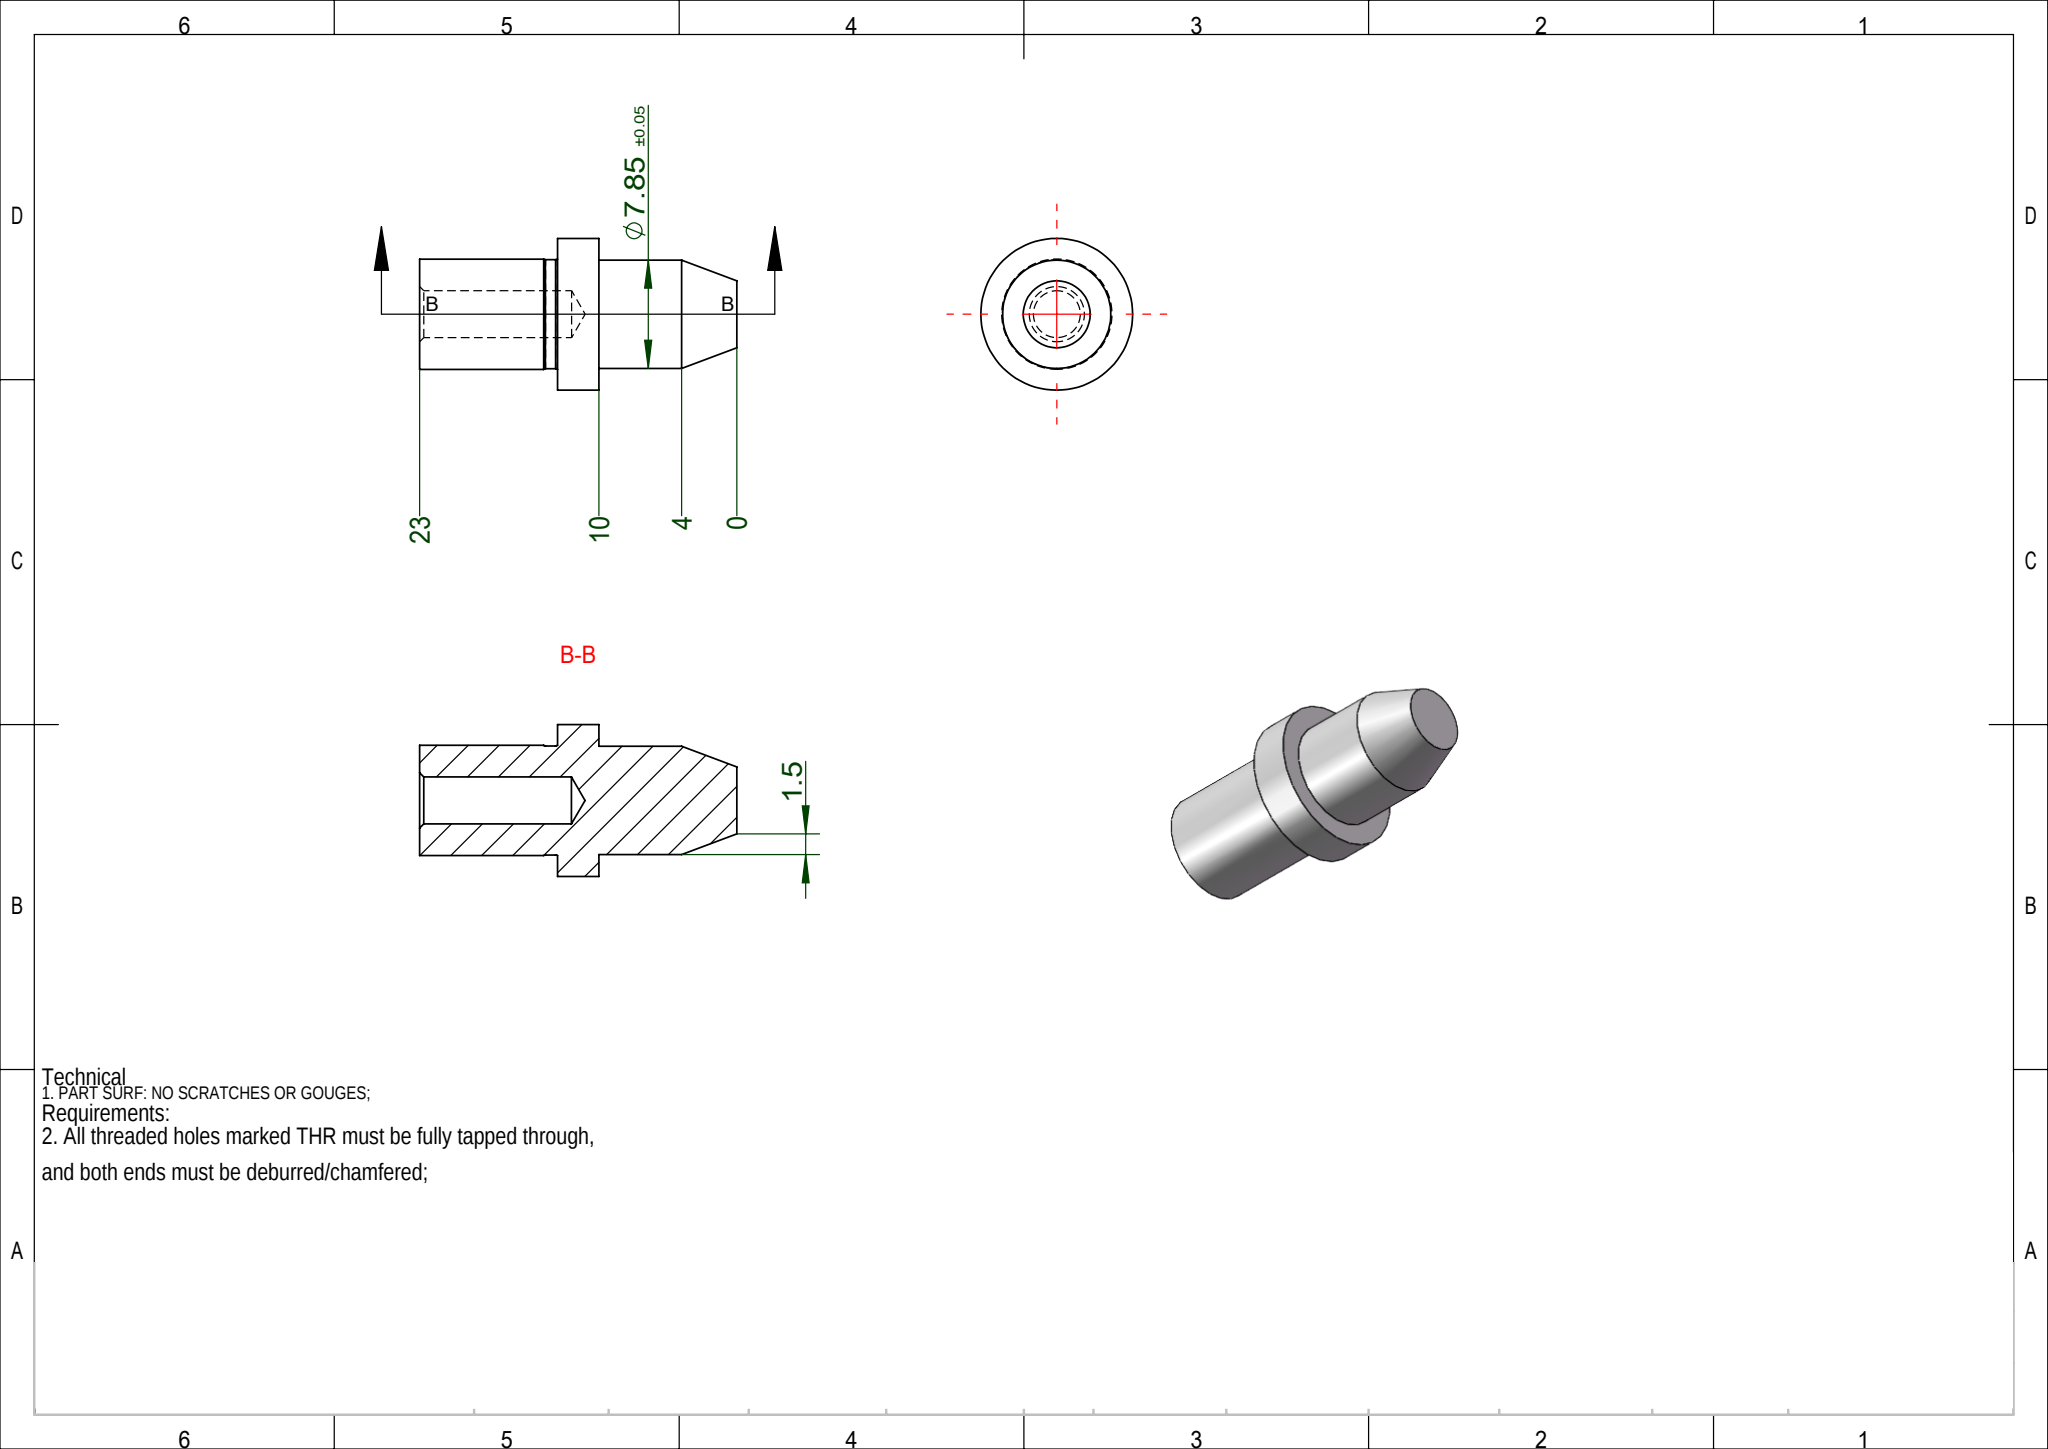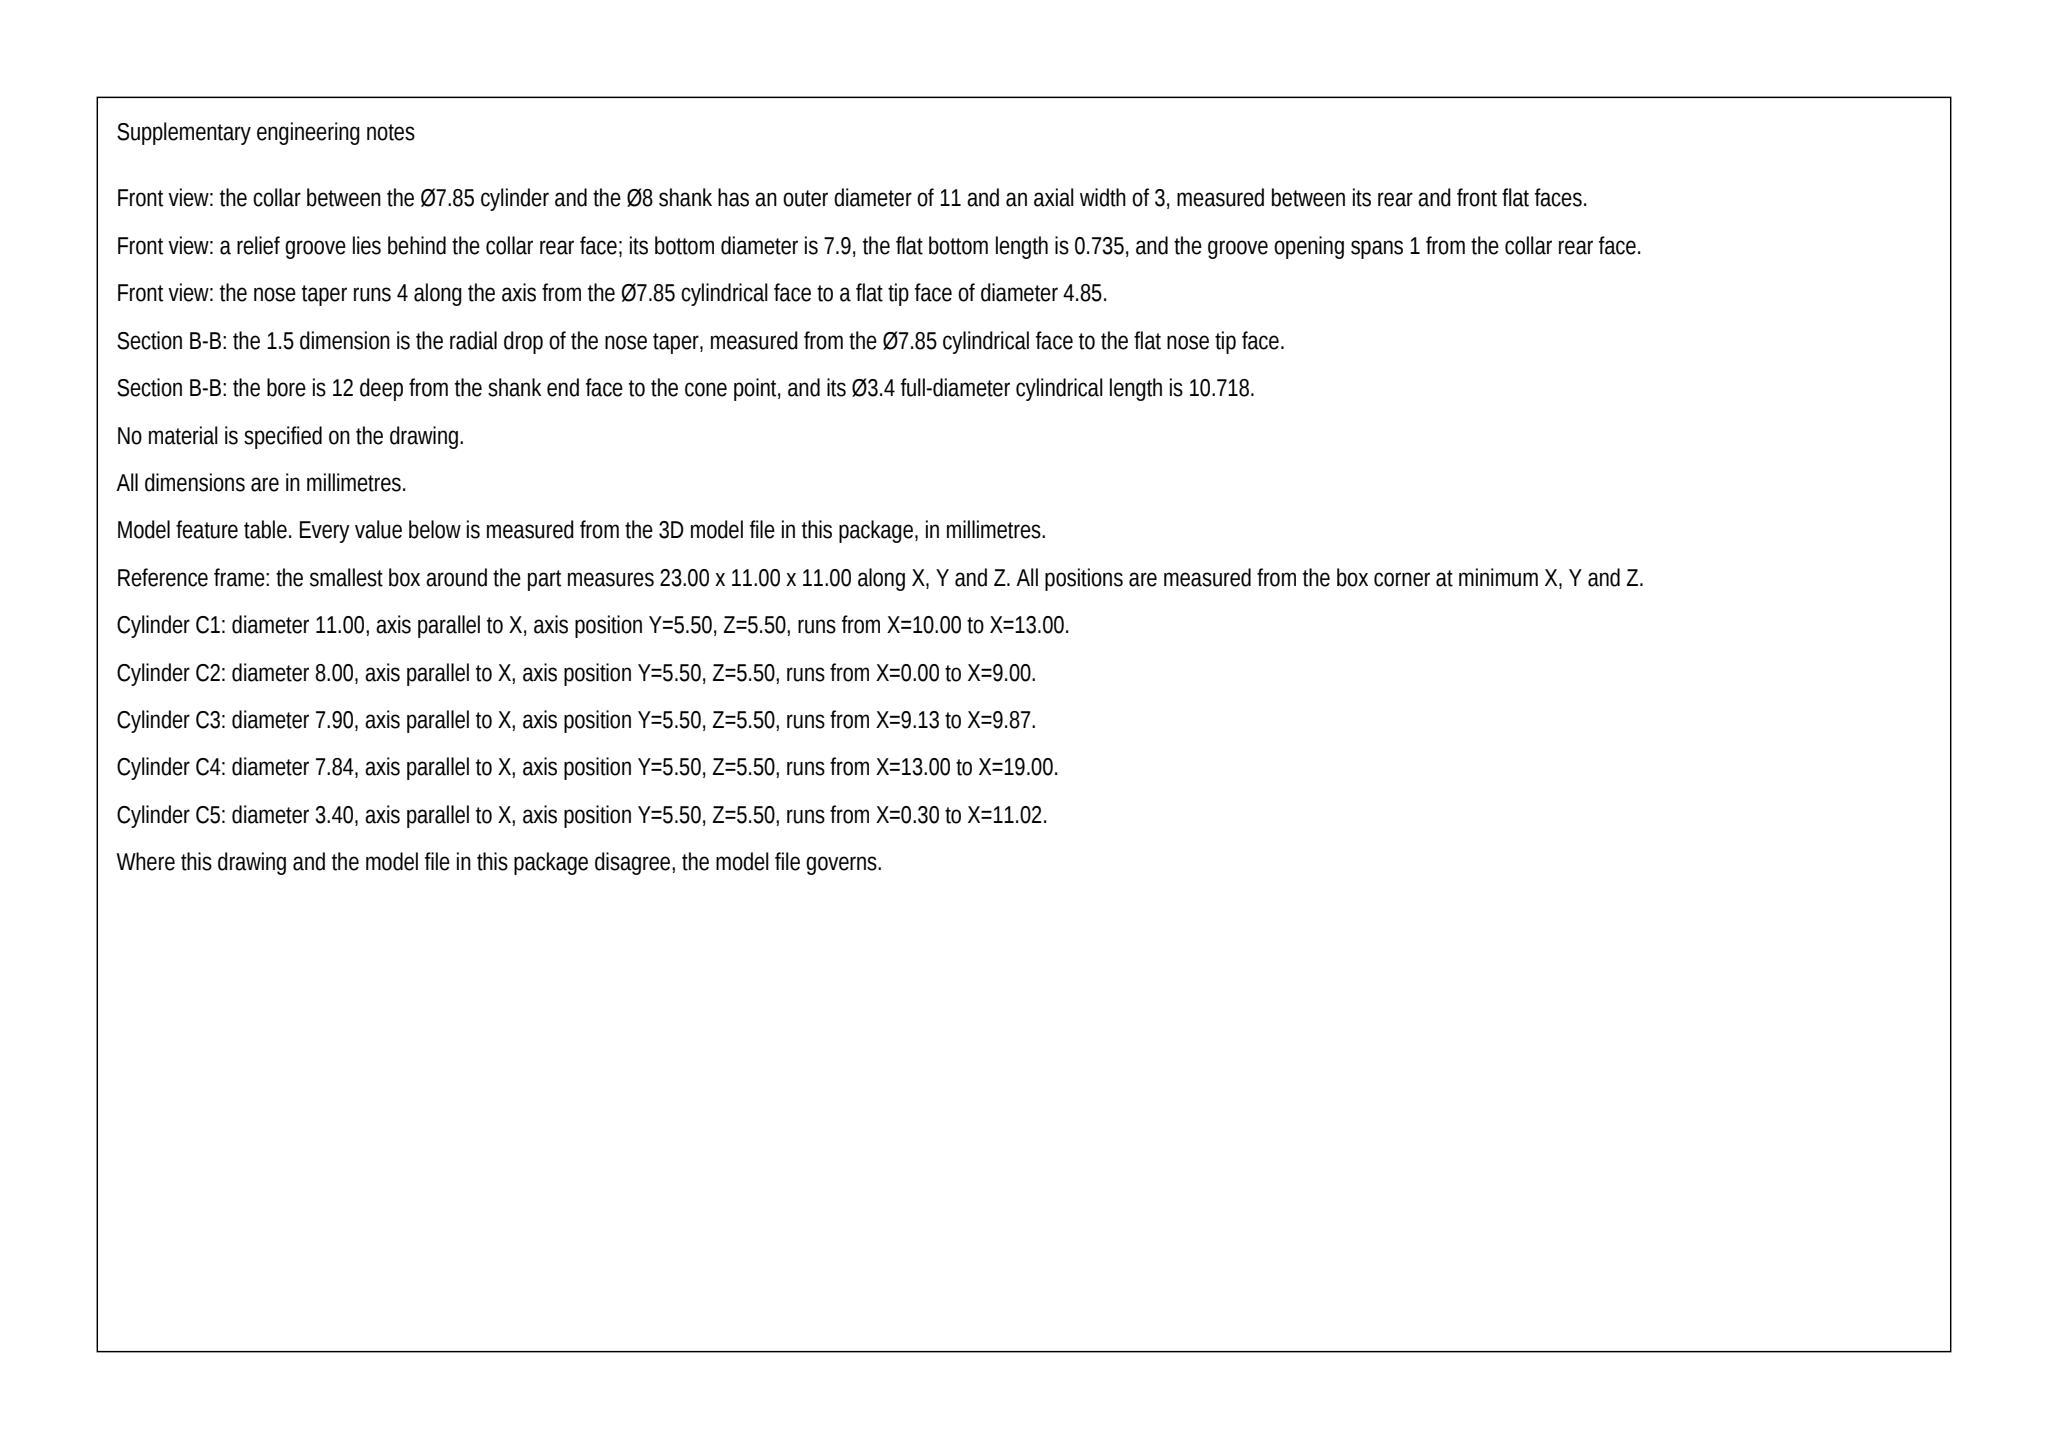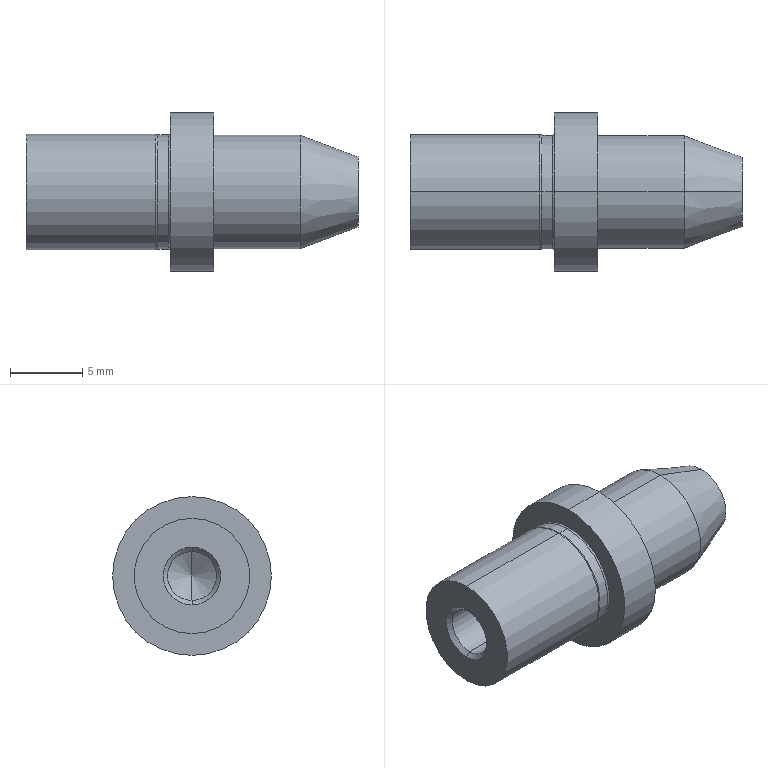Part | SolidWorks | mm | 1 solid | 24 faces | box 23 x 11 x 11 mm | volume 1103 mm3 | cylinder 10 | cone 6 | spline 4 | plane 4 | commonest cylinder face diameters 7.85 x2 8 x2 7.9 x2 3.4 x2 11 x2
Drawing notes:
Ø8 SHANK x 10 LG, 13 TO 23 FROM 0 DATUM | from the solid: cyl dia 8 on x-axis, L=9 + Ø7.9 groove 0.74; planes x=13 and x=23
Ø11 FLANGE x 3 WIDE, 10 TO 13 FROM 0 DATUM | from the solid: cyl dia 11, axis x, length 3.0; planes x=10 and x=13
Ø3.4 BORE DP 10.72 FROM LH END (23 DATUM) | from the solid: cyl dia 3.4, axis x, length 10.72, open at x=23 face
Ø3.4 BORE BOTTOM 120° INCL DRILL PT | from the solid: cone included angle 120.0, ref dia 3.4
RELIEF GROOVE Ø7.9 x 0.74 W AT FLANGE, 13 TO 13.74 | from the solid: cyl dia 7.9, axis x, length 0.74, adjacent flange face x=13
NOSE TIP: 90° CHAM TO Ø4 END FACE | from the solid: cone included angle 90.0, ref dia 4.0 at x=0 end plane
NOSE TAPER 41.1° INCL FROM Ø7.85 AT 4 TO TIP | from the solid: cone included angle 41.1, ref dia 7.85; Ø7.85 cyl ends at x=4
STEP:
#1=CARTESIAN_POINT('',(-3.868,0.,-3.95));
#2=VERTEX_POINT('',#1);
#3=CARTESIAN_POINT('',(-3.868,0.,3.95));
#4=VERTEX_POINT('',#3);
#5=CARTESIAN_POINT('',(-3.868,0.,0.));
#6=DIRECTION('',(1.,0.,0.));
#7=DIRECTION('',(0.,0.,1.));
#8=AXIS2_PLACEMENT_3D('',#5,#6,#7);
#9=CIRCLE('',#8,3.95);
#10=EDGE_CURVE('',#2,#4,#9,.T.);
#11=ORIENTED_EDGE('',*,*,#10,.F.);
#12=CARTESIAN_POINT('',(-4.,0.,-4.));
#13=VERTEX_POINT('',#12);
#14=CARTESIAN_POINT('',(-3.868,0.,-4.15));
#15=DIRECTION('',(0.,-1.,-0.));
#16=DIRECTION('',(0.,0.,-1.));
#17=AXIS2_PLACEMENT_3D('',#14,#15,#16);
#18=CIRCLE('',#17,0.2);
#19=EDGE_CURVE('',#2,#13,#18,.T.);
#20=ORIENTED_EDGE('',*,*,#19,.T.);
#21=CARTESIAN_POINT('',(-4.,0.,4.));
#22=VERTEX_POINT('',#21);
#23=CARTESIAN_POINT('',(-4.,0.,0.));
#24=DIRECTION('',(-1.,0.,0.));
#25=DIRECTION('',(0.,0.,-1.));
#26=AXIS2_PLACEMENT_3D('',#23,#24,#25);
#27=CIRCLE('',#26,4.);
#28=EDGE_CURVE('',#22,#13,#27,.T.);
#29=ORIENTED_EDGE('',*,*,#28,.F.);
#30=CARTESIAN_POINT('',(-3.868,0.,4.15));
#31=DIRECTION('',(0.,1.,0.));
#32=DIRECTION('',(0.,0.,1.));
#33=AXIS2_PLACEMENT_3D('',#30,#31,#32);
#34=CIRCLE('',#33,0.2);
#35=EDGE_CURVE('',#4,#22,#34,.T.);
#36=ORIENTED_EDGE('',*,*,#35,.F.);
#37=EDGE_LOOP('',(#11,#20,#29,#36));
#38=FACE_OUTER_BOUND('',#37,.T.);
#39=CARTESIAN_POINT('',(-3.868,0.,3.95));
#40=CARTESIAN_POINT('',(-3.868,7.9,3.95));
#41=CARTESIAN_POINT('',(-3.868,7.9,-3.95));
#42=CARTESIAN_POINT('',(-3.868,0.,-3.95));
#43=CARTESIAN_POINT('',(-3.917,0.,3.95));
#44=CARTESIAN_POINT('',(-3.917,7.9,3.95));
#45=CARTESIAN_POINT('',(-3.917,7.9,-3.95));
#46=CARTESIAN_POINT('',(-3.917,0.,-3.95));
#47=CARTESIAN_POINT('',(-3.963,0.,3.967));
#48=CARTESIAN_POINT('',(-3.963,7.935,3.967));
#49=CARTESIAN_POINT('',(-3.963,7.935,-3.967));
#50=CARTESIAN_POINT('',(-3.963,0.,-3.967));
#51=CARTESIAN_POINT('',(-4.,0.,4.));
#52=CARTESIAN_POINT('',(-4.,8.,4.));
#53=CARTESIAN_POINT('',(-4.,8.,-4.));
#54=CARTESIAN_POINT('',(-4.,0.,-4.));
#55=(BOUNDED_SURFACE()B_SPLINE_SURFACE(3,3,((#39,#40,#41,#42),(#43,#44,#45,#46),(#47,#48,#49,#50),(#51,#52,#53,#54)),.UNSPECIFIED.,.F.,.F.,.T.)B_SPLINE_SURFACE_WITH_KNOTS((4,4),(4,4),(0.,1.),(0.,1.),.UNSPECIFIED.)GEOMETRIC_REPRESENTATION_ITEM()RATIONAL_B_SPLINE_SURFACE(((1.,0.3333,0.3333,1.),(0.9569,0.319,0.319,0.9569),(0.9569,0.319,0.319,0.9569),(1.,0.3333,0.3333,1.)))REPRESENTATION_ITEM('')SURFACE());
#56=ADVANCED_FACE('',(#38),#55,.F.);
#57=CARTESIAN_POINT('',(-3.,0.,-4.));
#58=VERTEX_POINT('',#57);
#59=CARTESIAN_POINT('',(-3.,0.,4.));
#60=VERTEX_POINT('',#59);
#61=CARTESIAN_POINT('',(-3.,0.,0.));
#62=DIRECTION('',(1.,0.,0.));
#63=DIRECTION('',(0.,0.,1.));
#64=AXIS2_PLACEMENT_3D('',#61,#62,#63);
#65=CIRCLE('',#64,4.);
#66=EDGE_CURVE('',#58,#60,#65,.T.);
#67=ORIENTED_EDGE('',*,*,#66,.F.);
#68=CARTESIAN_POINT('',(-3.132,0.,-3.95));
#69=VERTEX_POINT('',#68);
#70=CARTESIAN_POINT('',(-3.132,0.,-4.15));
#71=DIRECTION('',(0.,-1.,-0.));
#72=DIRECTION('',(0.,0.,-1.));
#73=AXIS2_PLACEMENT_3D('',#70,#71,#72);
#74=CIRCLE('',#73,0.2);
#75=EDGE_CURVE('',#58,#69,#74,.T.);
#76=ORIENTED_EDGE('',*,*,#75,.T.);
#77=CARTESIAN_POINT('',(-3.132,0.,3.95));
#78=VERTEX_POINT('',#77);
#79=CARTESIAN_POINT('',(-3.132,0.,0.));
#80=DIRECTION('',(-1.,0.,0.));
#81=DIRECTION('',(0.,0.,-1.));
#82=AXIS2_PLACEMENT_3D('',#79,#80,#81);
#83=CIRCLE('',#82,3.95);
#84=EDGE_CURVE('',#78,#69,#83,.T.);
#85=ORIENTED_EDGE('',*,*,#84,.F.);
#86=CARTESIAN_POINT('',(-3.132,0.,4.15));
#87=DIRECTION('',(0.,1.,0.));
#88=DIRECTION('',(0.,0.,1.));
#89=AXIS2_PLACEMENT_3D('',#86,#87,#88);
#90=CIRCLE('',#89,0.2);
#91=EDGE_CURVE('',#60,#78,#90,.T.);
#92=ORIENTED_EDGE('',*,*,#91,.F.);
#93=EDGE_LOOP('',(#67,#76,#85,#92));
#94=FACE_OUTER_BOUND('',#93,.T.);
#95=CARTESIAN_POINT('',(-3.,0.,4.));
#96=CARTESIAN_POINT('',(-3.,8.,4.));
#97=CARTESIAN_POINT('',(-3.,8.,-4.));
#98=CARTESIAN_POINT('',(-3.,0.,-4.));
#99=CARTESIAN_POINT('',(-3.037,0.,3.967));
#100=CARTESIAN_POINT('',(-3.037,7.935,3.967));
#101=CARTESIAN_POINT('',(-3.037,7.935,-3.967));
#102=CARTESIAN_POINT('',(-3.037,0.,-3.967));
#103=CARTESIAN_POINT('',(-3.083,0.,3.95));
#104=CARTESIAN_POINT('',(-3.083,7.9,3.95));
#105=CARTESIAN_POINT('',(-3.083,7.9,-3.95));
#106=CARTESIAN_POINT('',(-3.083,0.,-3.95));
#107=CARTESIAN_POINT('',(-3.132,0.,3.95));
#108=CARTESIAN_POINT('',(-3.132,7.9,3.95));
#109=CARTESIAN_POINT('',(-3.132,7.9,-3.95));
#110=CARTESIAN_POINT('',(-3.132,0.,-3.95));
#111=(BOUNDED_SURFACE()B_SPLINE_SURFACE(3,3,((#95,#96,#97,#98),(#99,#100,#101,#102),(#103,#104,#105,#106),(#107,#108,#109,#110)),.UNSPECIFIED.,.F.,.F.,.T.)B_SPLINE_SURFACE_WITH_KNOTS((4,4),(4,4),(0.,1.),(0.,1.),.UNSPECIFIED.)GEOMETRIC_REPRESENTATION_ITEM()RATIONAL_B_SPLINE_SURFACE(((1.,0.3333,0.3333,1.),(0.9569,0.319,0.319,0.9569),(0.9569,0.319,0.319,0.9569),(1.,0.3333,0.3333,1.)))REPRESENTATION_ITEM('')SURFACE());
#112=ADVANCED_FACE('',(#94),#111,.F.);
#113=CARTESIAN_POINT('',(10.,-0.,-2.425));
#114=VERTEX_POINT('',#113);
#115=CARTESIAN_POINT('',(10.,-0.,2.425));
#116=VERTEX_POINT('',#115);
#117=CARTESIAN_POINT('',(10.,-0.,0.));
#118=DIRECTION('',(1.,0.,0.));
#119=DIRECTION('',(0.,-1.,0.));
#120=AXIS2_PLACEMENT_3D('',#117,#118,#119);
#121=CIRCLE('',#120,2.425);
#122=EDGE_CURVE('',#114,#116,#121,.T.);
#123=ORIENTED_EDGE('',*,*,#122,.F.);
#124=CARTESIAN_POINT('',(6.,-0.,-3.925));
#125=VERTEX_POINT('',#124);
#126=CARTESIAN_POINT('',(6.,-0.,-3.925));
#127=DIRECTION('',(-0.9363,0.,-0.3511));
#128=VECTOR('',#127,1000.);
#129=LINE('',#126,#128);
#130=EDGE_CURVE('',#114,#125,#129,.T.);
#131=ORIENTED_EDGE('',*,*,#130,.T.);
#132=CARTESIAN_POINT('',(6.,-0.,3.925));
#133=VERTEX_POINT('',#132);
#134=CARTESIAN_POINT('',(6.,-0.,0.));
#135=DIRECTION('',(-1.,0.,0.));
#136=DIRECTION('',(0.,0.,1.));
#137=AXIS2_PLACEMENT_3D('',#134,#135,#136);
#138=CIRCLE('',#137,3.925);
#139=EDGE_CURVE('',#133,#125,#138,.T.);
#140=ORIENTED_EDGE('',*,*,#139,.F.);
#141=CARTESIAN_POINT('',(6.,-0.,3.925));
#142=DIRECTION('',(-0.9363,0.,0.3511));
#143=VECTOR('',#142,1000.);
#144=LINE('',#141,#143);
#145=EDGE_CURVE('',#116,#133,#144,.T.);
#146=ORIENTED_EDGE('',*,*,#145,.F.);
#147=EDGE_LOOP('',(#123,#131,#140,#146));
#148=FACE_OUTER_BOUND('',#147,.T.);
#149=CARTESIAN_POINT('',(6.,-0.,0.));
#150=DIRECTION('',(-1.,0.,0.));
#151=DIRECTION('',(0.,0.,1.));
#152=AXIS2_PLACEMENT_3D('',#149,#150,#151);
#153=CONICAL_SURFACE('',#152,3.925,0.3588);
#154=ADVANCED_FACE('',(#148),#153,.T.);
#155=ORIENTED_EDGE('',*,*,#139,.T.);
#156=CARTESIAN_POINT('',(0.,-0.,-3.925));
#157=VERTEX_POINT('',#156);
#158=CARTESIAN_POINT('',(15.,-0.,-3.925));
#159=DIRECTION('',(-1.,0.,0.));
#160=VECTOR('',#159,1000.);
#161=LINE('',#158,#160);
#162=EDGE_CURVE('',#125,#157,#161,.T.);
#163=ORIENTED_EDGE('',*,*,#162,.T.);
#164=CARTESIAN_POINT('',(0.,-0.,3.925));
#165=VERTEX_POINT('',#164);
#166=CARTESIAN_POINT('',(0.,-0.,0.));
#167=DIRECTION('',(1.,0.,0.));
#168=DIRECTION('',(0.,0.,-1.));
#169=AXIS2_PLACEMENT_3D('',#166,#167,#168);
#170=CIRCLE('',#169,3.925);
#171=EDGE_CURVE('',#157,#165,#170,.T.);
#172=ORIENTED_EDGE('',*,*,#171,.T.);
#173=CARTESIAN_POINT('',(15.,-0.,3.925));
#174=DIRECTION('',(-1.,0.,0.));
#175=VECTOR('',#174,1000.);
#176=LINE('',#173,#175);
#177=EDGE_CURVE('',#133,#165,#176,.T.);
#178=ORIENTED_EDGE('',*,*,#177,.F.);
#179=EDGE_LOOP('',(#155,#163,#172,#178));
#180=FACE_OUTER_BOUND('',#179,.T.);
#181=CARTESIAN_POINT('',(15.,-0.,0.));
#182=DIRECTION('',(-1.,0.,0.));
#183=DIRECTION('',(0.,0.,1.));
#184=AXIS2_PLACEMENT_3D('',#181,#182,#183);
#185=CYLINDRICAL_SURFACE('',#184,3.925);
#186=ADVANCED_FACE('',(#180),#185,.T.);
#187=CARTESIAN_POINT('',(-13.,0.,-4.));
#188=VERTEX_POINT('',#187);
#189=CARTESIAN_POINT('',(-13.,0.,4.));
#190=VERTEX_POINT('',#189);
#191=CARTESIAN_POINT('',(-13.,0.,0.));
#192=DIRECTION('',(1.,0.,0.));
#193=DIRECTION('',(0.,0.,-1.));
#194=AXIS2_PLACEMENT_3D('',#191,#192,#193);
#195=CIRCLE('',#194,4.);
#196=EDGE_CURVE('',#188,#190,#195,.T.);
#197=ORIENTED_EDGE('',*,*,#196,.T.);
#198=CARTESIAN_POINT('',(-8.5,0.,4.));
#199=DIRECTION('',(1.,0.,0.));
#200=VECTOR('',#199,1000.);
#201=LINE('',#198,#200);
#202=EDGE_CURVE('',#190,#22,#201,.T.);
#203=ORIENTED_EDGE('',*,*,#202,.T.);
#204=ORIENTED_EDGE('',*,*,#28,.T.);
#205=CARTESIAN_POINT('',(-8.5,0.,-4.));
#206=DIRECTION('',(1.,0.,0.));
#207=VECTOR('',#206,1000.);
#208=LINE('',#205,#207);
#209=EDGE_CURVE('',#188,#13,#208,.T.);
#210=ORIENTED_EDGE('',*,*,#209,.F.);
#211=EDGE_LOOP('',(#197,#203,#204,#210));
#212=FACE_OUTER_BOUND('',#211,.T.);
#213=CARTESIAN_POINT('',(-8.5,0.,0.));
#214=DIRECTION('',(1.,0.,0.));
#215=DIRECTION('',(0.,0.,-1.));
#216=AXIS2_PLACEMENT_3D('',#213,#214,#215);
#217=CYLINDRICAL_SURFACE('',#216,4.);
#218=ADVANCED_FACE('',(#212),#217,.T.);
#219=ORIENTED_EDGE('',*,*,#10,.T.);
#220=CARTESIAN_POINT('',(-3.5,0.,3.95));
#221=DIRECTION('',(1.,0.,0.));
#222=VECTOR('',#221,1000.);
#223=LINE('',#220,#222);
#224=EDGE_CURVE('',#4,#78,#223,.T.);
#225=ORIENTED_EDGE('',*,*,#224,.T.);
#226=ORIENTED_EDGE('',*,*,#84,.T.);
#227=CARTESIAN_POINT('',(-3.5,0.,-3.95));
#228=DIRECTION('',(1.,0.,0.));
#229=VECTOR('',#228,1000.);
#230=LINE('',#227,#229);
#231=EDGE_CURVE('',#2,#69,#230,.T.);
#232=ORIENTED_EDGE('',*,*,#231,.F.);
#233=EDGE_LOOP('',(#219,#225,#226,#232));
#234=FACE_OUTER_BOUND('',#233,.T.);
#235=CARTESIAN_POINT('',(-3.5,0.,0.));
#236=DIRECTION('',(1.,0.,0.));
#237=DIRECTION('',(0.,0.,-1.));
#238=AXIS2_PLACEMENT_3D('',#235,#236,#237);
#239=CYLINDRICAL_SURFACE('',#238,3.95);
#240=ADVANCED_FACE('',(#234),#239,.T.);
#241=CARTESIAN_POINT('',(-12.7,0.,-1.7));
#242=VERTEX_POINT('',#241);
#243=CARTESIAN_POINT('',(-12.7,0.,1.7));
#244=VERTEX_POINT('',#243);
#245=CARTESIAN_POINT('',(-12.7,0.,0.));
#246=DIRECTION('',(-1.,0.,0.));
#247=DIRECTION('',(0.,1.,-0.));
#248=AXIS2_PLACEMENT_3D('',#245,#246,#247);
#249=CIRCLE('',#248,1.7);
#250=EDGE_CURVE('',#242,#244,#249,.T.);
#251=ORIENTED_EDGE('',*,*,#250,.F.);
#252=CARTESIAN_POINT('',(-13.,0.,-2.));
#253=VERTEX_POINT('',#252);
#254=CARTESIAN_POINT('',(-13.,0.,-2.));
#255=DIRECTION('',(-0.7071,0.,-0.7071));
#256=VECTOR('',#255,1000.);
#257=LINE('',#254,#256);
#258=EDGE_CURVE('',#242,#253,#257,.T.);
#259=ORIENTED_EDGE('',*,*,#258,.T.);
#260=CARTESIAN_POINT('',(-13.,0.,2.));
#261=VERTEX_POINT('',#260);
#262=CARTESIAN_POINT('',(-13.,0.,0.));
#263=DIRECTION('',(1.,0.,0.));
#264=DIRECTION('',(0.,0.,1.));
#265=AXIS2_PLACEMENT_3D('',#262,#263,#264);
#266=CIRCLE('',#265,2.);
#267=EDGE_CURVE('',#261,#253,#266,.T.);
#268=ORIENTED_EDGE('',*,*,#267,.F.);
#269=CARTESIAN_POINT('',(-13.,0.,2.));
#270=DIRECTION('',(-0.7071,0.,0.7071));
#271=VECTOR('',#270,1000.);
#272=LINE('',#269,#271);
#273=EDGE_CURVE('',#244,#261,#272,.T.);
#274=ORIENTED_EDGE('',*,*,#273,.F.);
#275=EDGE_LOOP('',(#251,#259,#268,#274));
#276=FACE_OUTER_BOUND('',#275,.T.);
#277=CARTESIAN_POINT('',(-13.,0.,0.));
#278=DIRECTION('',(-1.,0.,0.));
#279=DIRECTION('',(0.,0.,1.));
#280=AXIS2_PLACEMENT_3D('',#277,#278,#279);
#281=CONICAL_SURFACE('',#280,2.,0.7854);
#282=ADVANCED_FACE('',(#276),#281,.F.);
#283=ORIENTED_EDGE('',*,*,#250,.T.);
#284=CARTESIAN_POINT('',(-1.981,0.,1.7));
#285=VERTEX_POINT('',#284);
#286=CARTESIAN_POINT('',(-7.491,0.,1.7));
#287=DIRECTION('',(1.,0.,0.));
#288=VECTOR('',#287,1000.);
#289=LINE('',#286,#288);
#290=EDGE_CURVE('',#244,#285,#289,.T.);
#291=ORIENTED_EDGE('',*,*,#290,.T.);
#292=CARTESIAN_POINT('',(-1.981,0.,-1.7));
#293=VERTEX_POINT('',#292);
#294=CARTESIAN_POINT('',(-1.981,0.,0.));
#295=DIRECTION('',(-1.,0.,0.));
#296=DIRECTION('',(0.,0.,-1.));
#297=AXIS2_PLACEMENT_3D('',#294,#295,#296);
#298=CIRCLE('',#297,1.7);
#299=EDGE_CURVE('',#293,#285,#298,.T.);
#300=ORIENTED_EDGE('',*,*,#299,.F.);
#301=CARTESIAN_POINT('',(-7.491,0.,-1.7));
#302=DIRECTION('',(1.,0.,0.));
#303=VECTOR('',#302,1000.);
#304=LINE('',#301,#303);
#305=EDGE_CURVE('',#242,#293,#304,.T.);
#306=ORIENTED_EDGE('',*,*,#305,.F.);
#307=EDGE_LOOP('',(#283,#291,#300,#306));
#308=FACE_OUTER_BOUND('',#307,.T.);
#309=CARTESIAN_POINT('',(-7.491,0.,0.));
#310=DIRECTION('',(1.,0.,0.));
#311=DIRECTION('',(0.,0.,-1.));
#312=AXIS2_PLACEMENT_3D('',#309,#310,#311);
#313=CYLINDRICAL_SURFACE('',#312,1.7);
#314=ADVANCED_FACE('',(#308),#313,.F.);
#315=CARTESIAN_POINT('',(-1.,0.,-0.));
#316=VERTEX_POINT('',#315);
#317=CARTESIAN_POINT('',(-1.981,0.,1.7));
#318=DIRECTION('',(-0.5,0.,0.866));
#319=VECTOR('',#318,1000.);
#320=LINE('',#317,#319);
#321=EDGE_CURVE('',#316,#285,#320,.T.);
#322=ORIENTED_EDGE('',*,*,#321,.F.);
#323=CARTESIAN_POINT('',(-1.981,0.,-1.7));
#324=DIRECTION('',(-0.5,0.,-0.866));
#325=VECTOR('',#324,1000.);
#326=LINE('',#323,#325);
#327=EDGE_CURVE('',#316,#293,#326,.T.);
#328=ORIENTED_EDGE('',*,*,#327,.T.);
#329=ORIENTED_EDGE('',*,*,#299,.T.);
#330=EDGE_LOOP('',(#322,#328,#329));
#331=FACE_OUTER_BOUND('',#330,.T.);
#332=CARTESIAN_POINT('',(-1.981,0.,0.));
#333=DIRECTION('',(-1.,0.,0.));
#334=DIRECTION('',(0.,0.,1.));
#335=AXIS2_PLACEMENT_3D('',#332,#333,#334);
#336=CONICAL_SURFACE('',#335,1.7,1.047);
#337=ADVANCED_FACE('',(#331),#336,.F.);
#338=CARTESIAN_POINT('',(-3.,0.,5.5));
#339=VERTEX_POINT('',#338);
#340=CARTESIAN_POINT('',(-3.,0.,-5.5));
#341=VERTEX_POINT('',#340);
#342=CARTESIAN_POINT('',(-3.,0.,0.));
#343=DIRECTION('',(-1.,0.,0.));
#344=DIRECTION('',(0.,0.,-1.));
#345=AXIS2_PLACEMENT_3D('',#342,#343,#344);
#346=CIRCLE('',#345,5.5);
#347=EDGE_CURVE('',#339,#341,#346,.T.);
#348=ORIENTED_EDGE('',*,*,#347,.F.);
#349=CARTESIAN_POINT('',(0.,0.,5.5));
#350=VERTEX_POINT('',#349);
#351=CARTESIAN_POINT('',(-1.5,0.,5.5));
#352=DIRECTION('',(1.,0.,0.));
#353=VECTOR('',#352,1000.);
#354=LINE('',#351,#353);
#355=EDGE_CURVE('',#339,#350,#354,.T.);
#356=ORIENTED_EDGE('',*,*,#355,.T.);
#357=CARTESIAN_POINT('',(0.,0.,-5.5));
#358=VERTEX_POINT('',#357);
#359=CARTESIAN_POINT('',(0.,0.,0.));
#360=DIRECTION('',(-1.,0.,0.));
#361=DIRECTION('',(0.,0.,-1.));
#362=AXIS2_PLACEMENT_3D('',#359,#360,#361);
#363=CIRCLE('',#362,5.5);
#364=EDGE_CURVE('',#350,#358,#363,.T.);
#365=ORIENTED_EDGE('',*,*,#364,.T.);
#366=CARTESIAN_POINT('',(-1.5,0.,-5.5));
#367=DIRECTION('',(1.,0.,0.));
#368=VECTOR('',#367,1000.);
#369=LINE('',#366,#368);
#370=EDGE_CURVE('',#341,#358,#369,.T.);
#371=ORIENTED_EDGE('',*,*,#370,.F.);
#372=EDGE_LOOP('',(#348,#356,#365,#371));
#373=FACE_OUTER_BOUND('',#372,.T.);
#374=CARTESIAN_POINT('',(-1.5,0.,0.));
#375=DIRECTION('',(1.,0.,0.));
#376=DIRECTION('',(0.,0.,-1.));
#377=AXIS2_PLACEMENT_3D('',#374,#375,#376);
#378=CYLINDRICAL_SURFACE('',#377,5.5);
#379=ADVANCED_FACE('',(#373),#378,.T.);
#380=ORIENTED_EDGE('',*,*,#202,.F.);
#381=CARTESIAN_POINT('',(-13.,0.,0.));
#382=DIRECTION('',(1.,0.,0.));
#383=DIRECTION('',(0.,0.,-1.));
#384=AXIS2_PLACEMENT_3D('',#381,#382,#383);
#385=CIRCLE('',#384,4.);
#386=EDGE_CURVE('',#190,#188,#385,.T.);
#387=ORIENTED_EDGE('',*,*,#386,.T.);
#388=ORIENTED_EDGE('',*,*,#209,.T.);
#389=CARTESIAN_POINT('',(-4.,0.,0.));
#390=DIRECTION('',(-1.,0.,0.));
#391=DIRECTION('',(0.,0.,-1.));
#392=AXIS2_PLACEMENT_3D('',#389,#390,#391);
#393=CIRCLE('',#392,4.);
#394=EDGE_CURVE('',#13,#22,#393,.T.);
#395=ORIENTED_EDGE('',*,*,#394,.T.);
#396=EDGE_LOOP('',(#380,#387,#388,#395));
#397=FACE_OUTER_BOUND('',#396,.T.);
#398=CARTESIAN_POINT('',(-8.5,0.,0.));
#399=DIRECTION('',(1.,0.,0.));
#400=DIRECTION('',(0.,0.,-1.));
#401=AXIS2_PLACEMENT_3D('',#398,#399,#400);
#402=CYLINDRICAL_SURFACE('',#401,4.);
#403=ADVANCED_FACE('',(#397),#402,.T.);
#404=ORIENTED_EDGE('',*,*,#19,.F.);
#405=CARTESIAN_POINT('',(-3.868,0.,0.));
#406=DIRECTION('',(1.,0.,0.));
#407=DIRECTION('',(0.,0.,1.));
#408=AXIS2_PLACEMENT_3D('',#405,#406,#407);
#409=CIRCLE('',#408,3.95);
#410=EDGE_CURVE('',#4,#2,#409,.T.);
#411=ORIENTED_EDGE('',*,*,#410,.F.);
#412=ORIENTED_EDGE('',*,*,#35,.T.);
#413=ORIENTED_EDGE('',*,*,#394,.F.);
#414=EDGE_LOOP('',(#404,#411,#412,#413));
#415=FACE_OUTER_BOUND('',#414,.T.);
#416=CARTESIAN_POINT('',(-3.868,0.,-3.95));
#417=CARTESIAN_POINT('',(-3.868,-7.9,-3.95));
#418=CARTESIAN_POINT('',(-3.868,-7.9,3.95));
#419=CARTESIAN_POINT('',(-3.868,-0.,3.95));
#420=CARTESIAN_POINT('',(-3.917,0.,-3.95));
#421=CARTESIAN_POINT('',(-3.917,-7.9,-3.95));
#422=CARTESIAN_POINT('',(-3.917,-7.9,3.95));
#423=CARTESIAN_POINT('',(-3.917,-0.,3.95));
#424=CARTESIAN_POINT('',(-3.963,0.,-3.967));
#425=CARTESIAN_POINT('',(-3.963,-7.935,-3.967));
#426=CARTESIAN_POINT('',(-3.963,-7.935,3.967));
#427=CARTESIAN_POINT('',(-3.963,-0.,3.967));
#428=CARTESIAN_POINT('',(-4.,0.,-4.));
#429=CARTESIAN_POINT('',(-4.,-8.,-4.));
#430=CARTESIAN_POINT('',(-4.,-8.,4.));
#431=CARTESIAN_POINT('',(-4.,-0.,4.));
#432=(BOUNDED_SURFACE()B_SPLINE_SURFACE(3,3,((#416,#417,#418,#419),(#420,#421,#422,#423),(#424,#425,#426,#427),(#428,#429,#430,#431)),.UNSPECIFIED.,.F.,.F.,.T.)B_SPLINE_SURFACE_WITH_KNOTS((4,4),(4,4),(0.,1.),(0.,1.),.UNSPECIFIED.)GEOMETRIC_REPRESENTATION_ITEM()RATIONAL_B_SPLINE_SURFACE(((1.,0.3333,0.3333,1.),(0.9569,0.319,0.319,0.9569),(0.9569,0.319,0.319,0.9569),(1.,0.3333,0.3333,1.)))REPRESENTATION_ITEM('')SURFACE());
#433=ADVANCED_FACE('',(#415),#432,.F.);
#434=ORIENTED_EDGE('',*,*,#196,.F.);
#435=ORIENTED_EDGE('',*,*,#386,.F.);
#436=EDGE_LOOP('',(#434,#435));
#437=FACE_OUTER_BOUND('',#436,.T.);
#438=ORIENTED_EDGE('',*,*,#267,.T.);
#439=CARTESIAN_POINT('',(-13.,0.,0.));
#440=DIRECTION('',(1.,0.,0.));
#441=DIRECTION('',(0.,0.,1.));
#442=AXIS2_PLACEMENT_3D('',#439,#440,#441);
#443=CIRCLE('',#442,2.);
#444=EDGE_CURVE('',#253,#261,#443,.T.);
#445=ORIENTED_EDGE('',*,*,#444,.T.);
#446=EDGE_LOOP('',(#438,#445));
#447=FACE_BOUND('',#446,.T.);
#448=CARTESIAN_POINT('',(-13.,2.,-0.));
#449=DIRECTION('',(-1.,0.,0.));
#450=DIRECTION('',(0.,0.,1.));
#451=AXIS2_PLACEMENT_3D('',#448,#449,#450);
#452=PLANE('',#451);
#453=ADVANCED_FACE('',(#437,#447),#452,.T.);
#454=ORIENTED_EDGE('',*,*,#224,.F.);
#455=ORIENTED_EDGE('',*,*,#410,.T.);
#456=ORIENTED_EDGE('',*,*,#231,.T.);
#457=CARTESIAN_POINT('',(-3.132,0.,0.));
#458=DIRECTION('',(-1.,0.,0.));
#459=DIRECTION('',(0.,0.,-1.));
#460=AXIS2_PLACEMENT_3D('',#457,#458,#459);
#461=CIRCLE('',#460,3.95);
#462=EDGE_CURVE('',#69,#78,#461,.T.);
#463=ORIENTED_EDGE('',*,*,#462,.T.);
#464=EDGE_LOOP('',(#454,#455,#456,#463));
#465=FACE_OUTER_BOUND('',#464,.T.);
#466=CARTESIAN_POINT('',(-3.5,0.,0.));
#467=DIRECTION('',(1.,0.,0.));
#468=DIRECTION('',(0.,0.,-1.));
#469=AXIS2_PLACEMENT_3D('',#466,#467,#468);
#470=CYLINDRICAL_SURFACE('',#469,3.95);
#471=ADVANCED_FACE('',(#465),#470,.T.);
#472=ORIENTED_EDGE('',*,*,#258,.F.);
#473=CARTESIAN_POINT('',(-12.7,0.,0.));
#474=DIRECTION('',(-1.,0.,0.));
#475=DIRECTION('',(0.,1.,-0.));
#476=AXIS2_PLACEMENT_3D('',#473,#474,#475);
#477=CIRCLE('',#476,1.7);
#478=EDGE_CURVE('',#244,#242,#477,.T.);
#479=ORIENTED_EDGE('',*,*,#478,.F.);
#480=ORIENTED_EDGE('',*,*,#273,.T.);
#481=ORIENTED_EDGE('',*,*,#444,.F.);
#482=EDGE_LOOP('',(#472,#479,#480,#481));
#483=FACE_OUTER_BOUND('',#482,.T.);
#484=CARTESIAN_POINT('',(-13.,0.,0.));
#485=DIRECTION('',(-1.,0.,0.));
#486=DIRECTION('',(0.,0.,1.));
#487=AXIS2_PLACEMENT_3D('',#484,#485,#486);
#488=CONICAL_SURFACE('',#487,2.,0.7854);
#489=ADVANCED_FACE('',(#483),#488,.F.);
#490=ORIENTED_EDGE('',*,*,#75,.F.);
#491=CARTESIAN_POINT('',(-3.,0.,0.));
#492=DIRECTION('',(1.,0.,0.));
#493=DIRECTION('',(0.,0.,1.));
#494=AXIS2_PLACEMENT_3D('',#491,#492,#493);
#495=CIRCLE('',#494,4.);
#496=EDGE_CURVE('',#60,#58,#495,.T.);
#497=ORIENTED_EDGE('',*,*,#496,.F.);
#498=ORIENTED_EDGE('',*,*,#91,.T.);
#499=ORIENTED_EDGE('',*,*,#462,.F.);
#500=EDGE_LOOP('',(#490,#497,#498,#499));
#501=FACE_OUTER_BOUND('',#500,.T.);
#502=CARTESIAN_POINT('',(-3.,0.,-4.));
#503=CARTESIAN_POINT('',(-3.,-8.,-4.));
#504=CARTESIAN_POINT('',(-3.,-8.,4.));
#505=CARTESIAN_POINT('',(-3.,-0.,4.));
#506=CARTESIAN_POINT('',(-3.037,0.,-3.967));
#507=CARTESIAN_POINT('',(-3.037,-7.935,-3.967));
#508=CARTESIAN_POINT('',(-3.037,-7.935,3.967));
#509=CARTESIAN_POINT('',(-3.037,-0.,3.967));
#510=CARTESIAN_POINT('',(-3.083,0.,-3.95));
#511=CARTESIAN_POINT('',(-3.083,-7.9,-3.95));
#512=CARTESIAN_POINT('',(-3.083,-7.9,3.95));
#513=CARTESIAN_POINT('',(-3.083,-0.,3.95));
#514=CARTESIAN_POINT('',(-3.132,0.,-3.95));
#515=CARTESIAN_POINT('',(-3.132,-7.9,-3.95));
#516=CARTESIAN_POINT('',(-3.132,-7.9,3.95));
#517=CARTESIAN_POINT('',(-3.132,-0.,3.95));
#518=(BOUNDED_SURFACE()B_SPLINE_SURFACE(3,3,((#502,#503,#504,#505),(#506,#507,#508,#509),(#510,#511,#512,#513),(#514,#515,#516,#517)),.UNSPECIFIED.,.F.,.F.,.T.)B_SPLINE_SURFACE_WITH_KNOTS((4,4),(4,4),(0.,1.),(0.,1.),.UNSPECIFIED.)GEOMETRIC_REPRESENTATION_ITEM()RATIONAL_B_SPLINE_SURFACE(((1.,0.3333,0.3333,1.),(0.9569,0.319,0.319,0.9569),(0.9569,0.319,0.319,0.9569),(1.,0.3333,0.3333,1.)))REPRESENTATION_ITEM('')SURFACE());
#519=ADVANCED_FACE('',(#501),#518,.F.);
#520=ORIENTED_EDGE('',*,*,#290,.F.);
#521=ORIENTED_EDGE('',*,*,#478,.T.);
#522=ORIENTED_EDGE('',*,*,#305,.T.);
#523=CARTESIAN_POINT('',(-1.981,0.,0.));
#524=DIRECTION('',(-1.,0.,0.));
#525=DIRECTION('',(0.,0.,-1.));
#526=AXIS2_PLACEMENT_3D('',#523,#524,#525);
#527=CIRCLE('',#526,1.7);
#528=EDGE_CURVE('',#285,#293,#527,.T.);
#529=ORIENTED_EDGE('',*,*,#528,.F.);
#530=EDGE_LOOP('',(#520,#521,#522,#529));
#531=FACE_OUTER_BOUND('',#530,.T.);
#532=CARTESIAN_POINT('',(-7.491,0.,0.));
#533=DIRECTION('',(1.,0.,0.));
#534=DIRECTION('',(0.,0.,-1.));
#535=AXIS2_PLACEMENT_3D('',#532,#533,#534);
#536=CYLINDRICAL_SURFACE('',#535,1.7);
#537=ADVANCED_FACE('',(#531),#536,.F.);
#538=CARTESIAN_POINT('',(-3.,0.,0.));
#539=DIRECTION('',(-1.,0.,0.));
#540=DIRECTION('',(0.,0.,-1.));
#541=AXIS2_PLACEMENT_3D('',#538,#539,#540);
#542=CIRCLE('',#541,5.5);
#543=EDGE_CURVE('',#341,#339,#542,.T.);
#544=ORIENTED_EDGE('',*,*,#543,.T.);
#545=ORIENTED_EDGE('',*,*,#347,.T.);
#546=EDGE_LOOP('',(#544,#545));
#547=FACE_OUTER_BOUND('',#546,.T.);
#548=ORIENTED_EDGE('',*,*,#496,.T.);
#549=ORIENTED_EDGE('',*,*,#66,.T.);
#550=EDGE_LOOP('',(#548,#549));
#551=FACE_BOUND('',#550,.T.);
#552=CARTESIAN_POINT('',(-3.,4.75,-0.));
#553=DIRECTION('',(-1.,0.,0.));
#554=DIRECTION('',(0.,0.,1.));
#555=AXIS2_PLACEMENT_3D('',#552,#553,#554);
#556=PLANE('',#555);
#557=ADVANCED_FACE('',(#547,#551),#556,.T.);
#558=ORIENTED_EDGE('',*,*,#327,.F.);
#559=ORIENTED_EDGE('',*,*,#321,.T.);
#560=ORIENTED_EDGE('',*,*,#528,.T.);
#561=EDGE_LOOP('',(#558,#559,#560));
#562=FACE_OUTER_BOUND('',#561,.T.);
#563=CARTESIAN_POINT('',(-1.981,0.,0.));
#564=DIRECTION('',(-1.,0.,0.));
#565=DIRECTION('',(0.,0.,1.));
#566=AXIS2_PLACEMENT_3D('',#563,#564,#565);
#567=CONICAL_SURFACE('',#566,1.7,1.047);
#568=ADVANCED_FACE('',(#562),#567,.F.);
#569=ORIENTED_EDGE('',*,*,#355,.F.);
#570=ORIENTED_EDGE('',*,*,#543,.F.);
#571=ORIENTED_EDGE('',*,*,#370,.T.);
#572=CARTESIAN_POINT('',(0.,0.,0.));
#573=DIRECTION('',(-1.,0.,0.));
#574=DIRECTION('',(0.,0.,-1.));
#575=AXIS2_PLACEMENT_3D('',#572,#573,#574);
#576=CIRCLE('',#575,5.5);
#577=EDGE_CURVE('',#358,#350,#576,.T.);
#578=ORIENTED_EDGE('',*,*,#577,.T.);
#579=EDGE_LOOP('',(#569,#570,#571,#578));
#580=FACE_OUTER_BOUND('',#579,.T.);
#581=CARTESIAN_POINT('',(-1.5,0.,0.));
#582=DIRECTION('',(1.,0.,0.));
#583=DIRECTION('',(0.,0.,-1.));
#584=AXIS2_PLACEMENT_3D('',#581,#582,#583);
#585=CYLINDRICAL_SURFACE('',#584,5.5);
#586=ADVANCED_FACE('',(#580),#585,.T.);
#587=ORIENTED_EDGE('',*,*,#577,.F.);
#588=ORIENTED_EDGE('',*,*,#364,.F.);
#589=EDGE_LOOP('',(#587,#588));
#590=FACE_OUTER_BOUND('',#589,.T.);
#591=CARTESIAN_POINT('',(0.,-0.,0.));
#592=DIRECTION('',(1.,0.,0.));
#593=DIRECTION('',(0.,0.,-1.));
#594=AXIS2_PLACEMENT_3D('',#591,#592,#593);
#595=CIRCLE('',#594,3.925);
#596=EDGE_CURVE('',#165,#157,#595,.T.);
#597=ORIENTED_EDGE('',*,*,#596,.F.);
#598=ORIENTED_EDGE('',*,*,#171,.F.);
#599=EDGE_LOOP('',(#597,#598));
#600=FACE_BOUND('',#599,.T.);
#601=CARTESIAN_POINT('',(0.,2.75,-0.));
#602=DIRECTION('',(1.,0.,0.));
#603=DIRECTION('',(0.,0.,-1.));
#604=AXIS2_PLACEMENT_3D('',#601,#602,#603);
#605=PLANE('',#604);
#606=ADVANCED_FACE('',(#590,#600),#605,.T.);
#607=ORIENTED_EDGE('',*,*,#162,.F.);
#608=CARTESIAN_POINT('',(6.,-0.,0.));
#609=DIRECTION('',(-1.,0.,0.));
#610=DIRECTION('',(0.,0.,1.));
#611=AXIS2_PLACEMENT_3D('',#608,#609,#610);
#612=CIRCLE('',#611,3.925);
#613=EDGE_CURVE('',#125,#133,#612,.T.);
#614=ORIENTED_EDGE('',*,*,#613,.T.);
#615=ORIENTED_EDGE('',*,*,#177,.T.);
#616=ORIENTED_EDGE('',*,*,#596,.T.);
#617=EDGE_LOOP('',(#607,#614,#615,#616));
#618=FACE_OUTER_BOUND('',#617,.T.);
#619=CARTESIAN_POINT('',(15.,-0.,0.));
#620=DIRECTION('',(-1.,0.,0.));
#621=DIRECTION('',(0.,0.,1.));
#622=AXIS2_PLACEMENT_3D('',#619,#620,#621);
#623=CYLINDRICAL_SURFACE('',#622,3.925);
#624=ADVANCED_FACE('',(#618),#623,.T.);
#625=CARTESIAN_POINT('',(10.,-0.,0.));
#626=DIRECTION('',(1.,0.,0.));
#627=DIRECTION('',(0.,-1.,0.));
#628=AXIS2_PLACEMENT_3D('',#625,#626,#627);
#629=CIRCLE('',#628,2.425);
#630=EDGE_CURVE('',#116,#114,#629,.T.);
#631=ORIENTED_EDGE('',*,*,#630,.T.);
#632=ORIENTED_EDGE('',*,*,#122,.T.);
#633=EDGE_LOOP('',(#631,#632));
#634=FACE_OUTER_BOUND('',#633,.T.);
#635=CARTESIAN_POINT('',(10.,5.575,-5.5));
#636=DIRECTION('',(-1.,-0.,0.));
#637=DIRECTION('',(0.,-1.,0.));
#638=AXIS2_PLACEMENT_3D('',#635,#636,#637);
#639=PLANE('',#638);
#640=ADVANCED_FACE('',(#634),#639,.F.);
#641=ORIENTED_EDGE('',*,*,#130,.F.);
#642=ORIENTED_EDGE('',*,*,#630,.F.);
#643=ORIENTED_EDGE('',*,*,#145,.T.);
#644=ORIENTED_EDGE('',*,*,#613,.F.);
#645=EDGE_LOOP('',(#641,#642,#643,#644));
#646=FACE_OUTER_BOUND('',#645,.T.);
#647=CARTESIAN_POINT('',(6.,-0.,0.));
#648=DIRECTION('',(-1.,0.,0.));
#649=DIRECTION('',(0.,0.,1.));
#650=AXIS2_PLACEMENT_3D('',#647,#648,#649);
#651=CONICAL_SURFACE('',#650,3.925,0.3588);
#652=ADVANCED_FACE('',(#646),#651,.T.);
#653=CLOSED_SHELL('',(#56,#112,#154,#186,#218,#240,#282,#314,#337,#379,#403,#433,#453,#471,#489,#519,#537,#557,#568,#586,#606,#624,#640,#652));
#654=MANIFOLD_SOLID_BREP('',#653);
#655=CARTESIAN_POINT('',(0.,0.,0.));
#656=DIRECTION('',(0.,0.,1.));
#657=DIRECTION('',(1.,0.,0.));
#658=AXIS2_PLACEMENT_3D('',#655,#656,#657);
#659=(LENGTH_UNIT()NAMED_UNIT(*)SI_UNIT(.MILLI.,.METRE.));
#660=UNCERTAINTY_MEASURE_WITH_UNIT(LENGTH_MEASURE(0.00001),#659,'','');
#661=(NAMED_UNIT(*)PLANE_ANGLE_UNIT()SI_UNIT($,.RADIAN.));
#662=(NAMED_UNIT(*)SI_UNIT($,.STERADIAN.)SOLID_ANGLE_UNIT());
#663=(GEOMETRIC_REPRESENTATION_CONTEXT(3)GLOBAL_UNCERTAINTY_ASSIGNED_CONTEXT((#660))GLOBAL_UNIT_ASSIGNED_CONTEXT((#659,#661,#662))REPRESENTATION_CONTEXT('',''));
#664=ADVANCED_BREP_SHAPE_REPRESENTATION('',(#654,#658),#663);